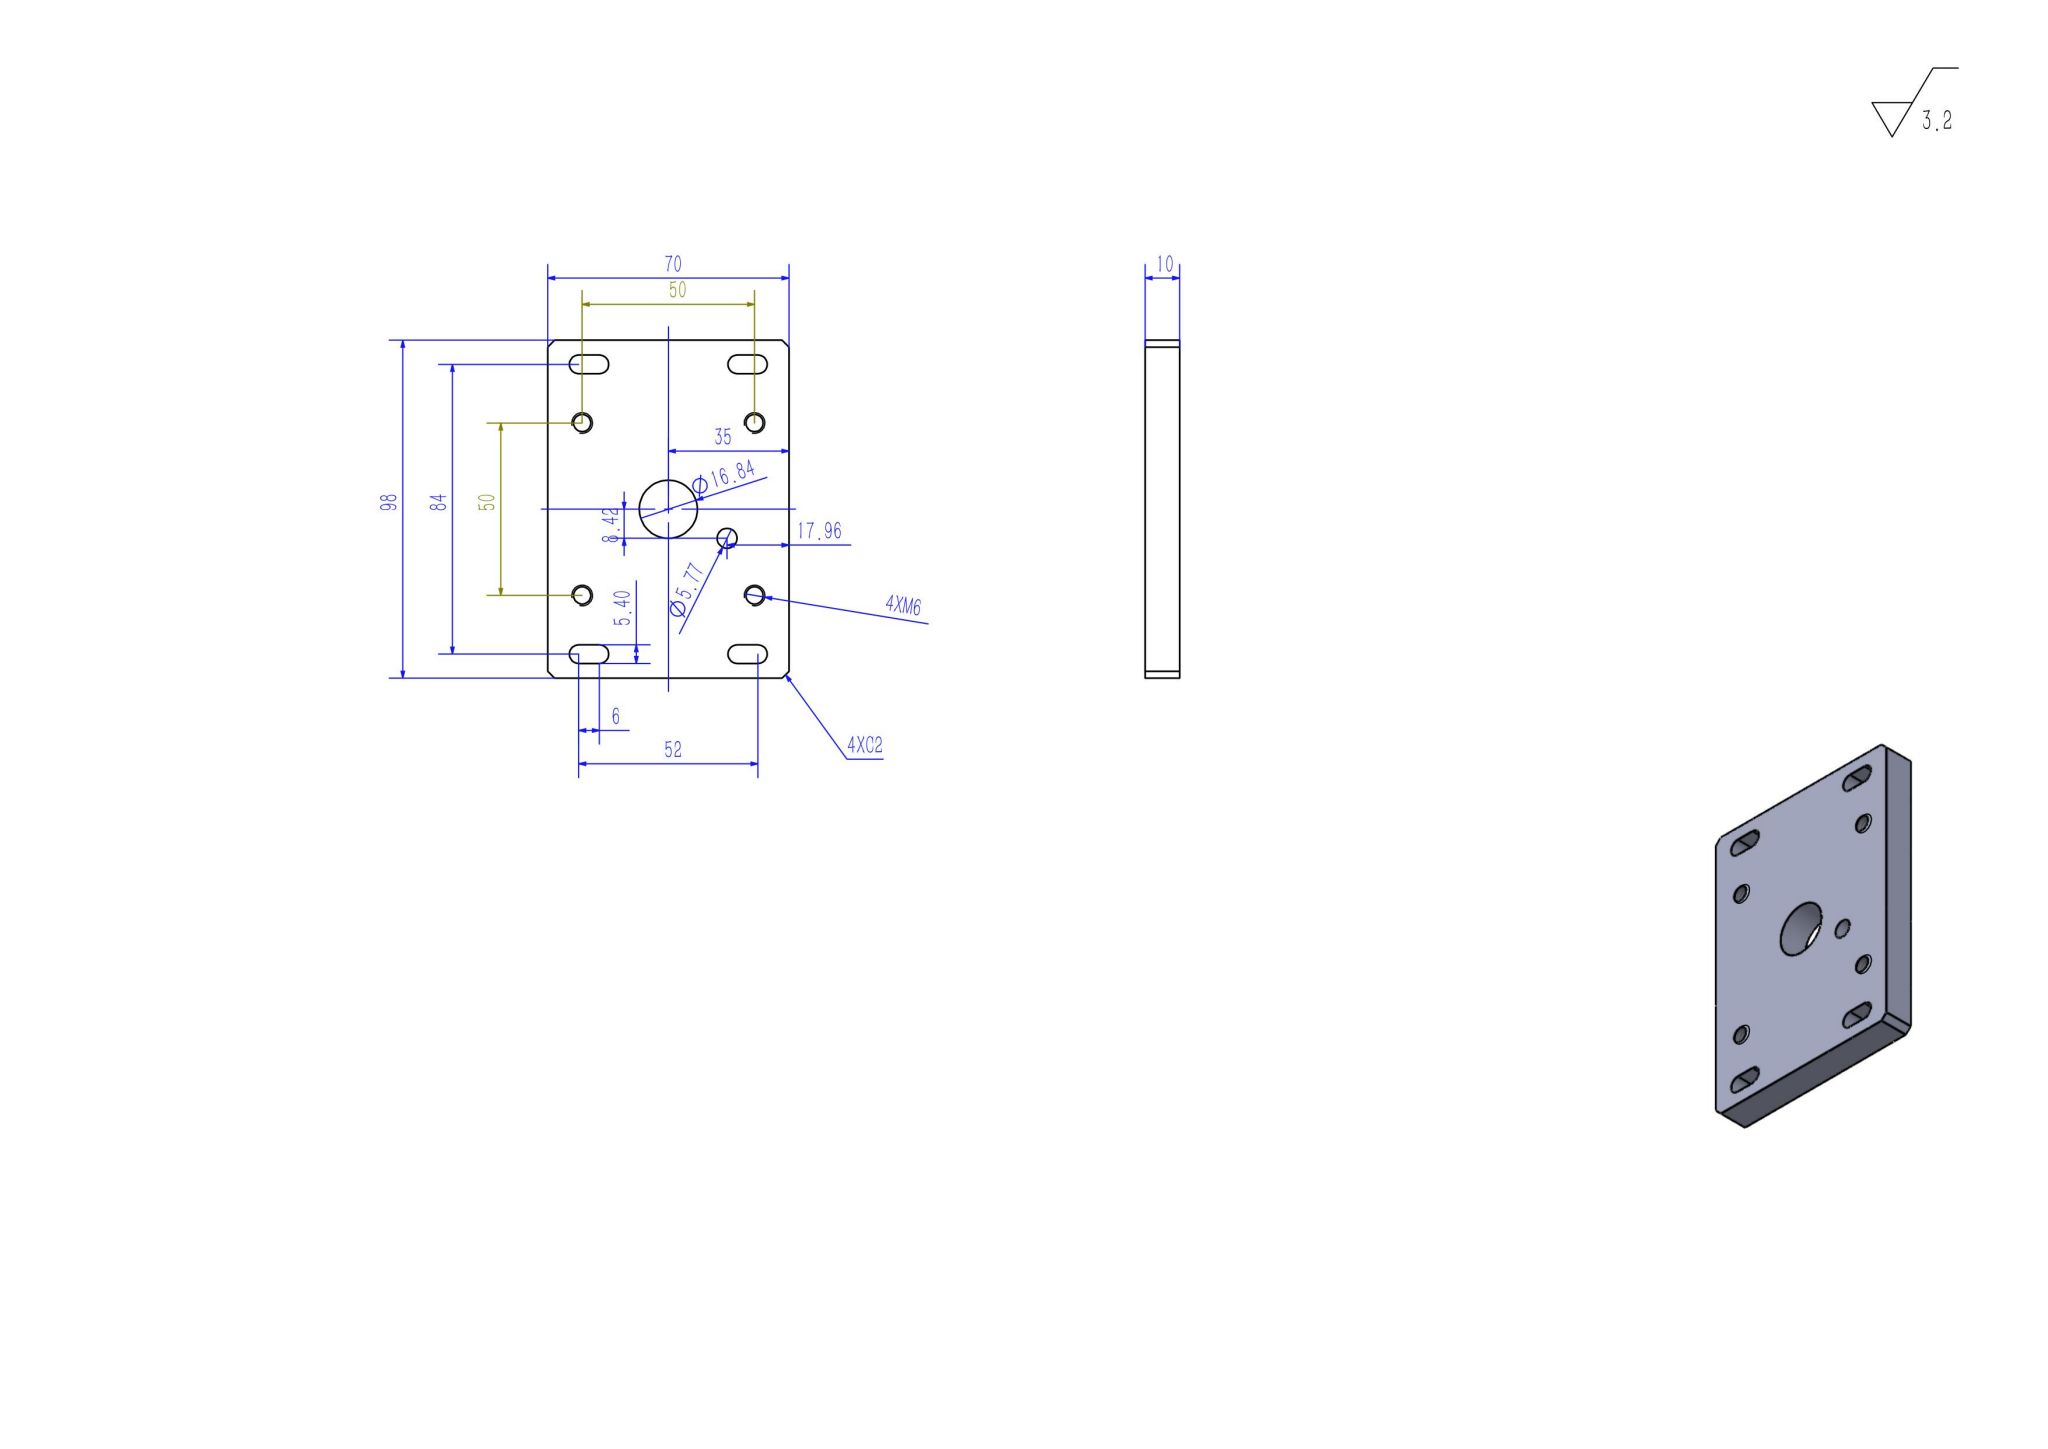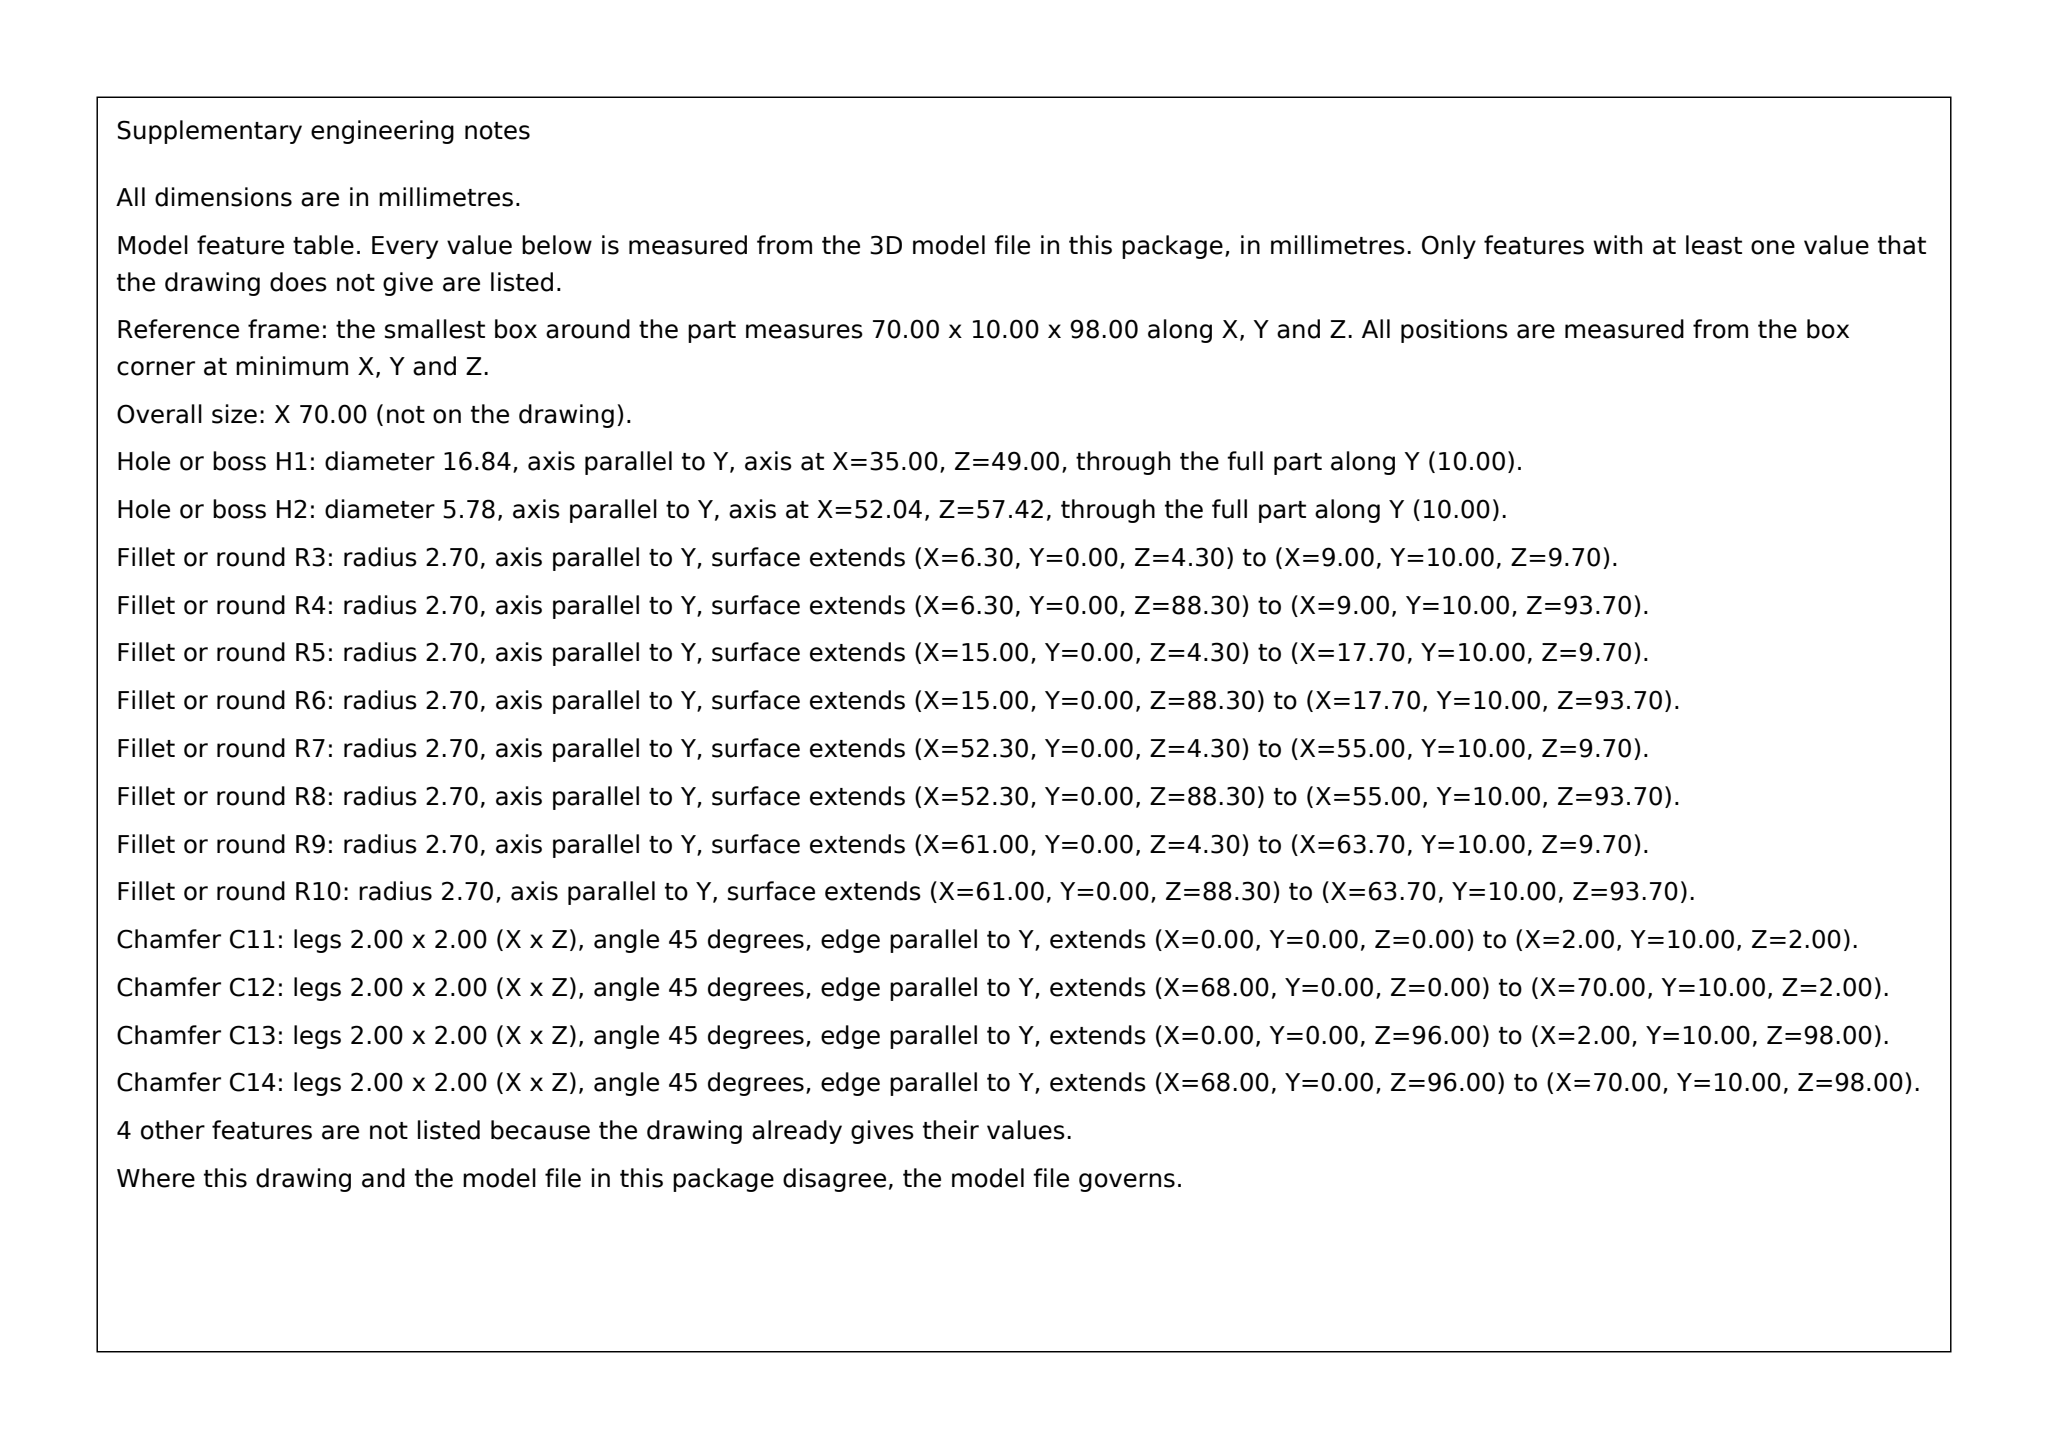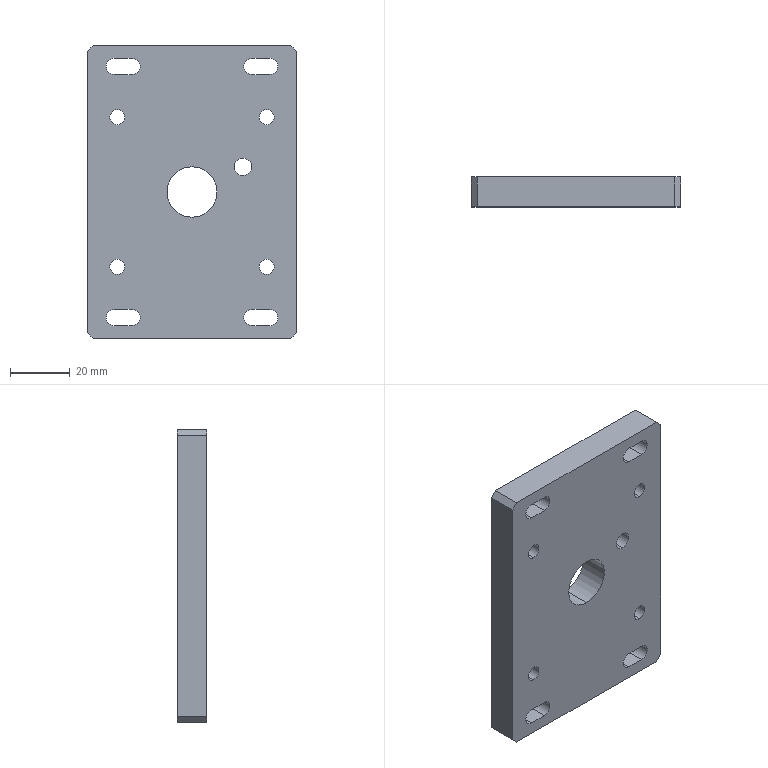Part | SolidWorks | mm | 1 solid | 38 faces | box 70 x 10 x 98 mm | volume 63034 mm3 | cylinder 20 | plane 18 | commonest cylinder face diameters 5 x8 5.4 x8 16.839 x2 5.77 x2
build123d program:
from build123d import *

# Parameters (mm, degrees)
SKETCH1_W             = 70
SKETCH1_H             = 98
BOSS_EXTRUDE1_DEPTH   = 10
M6_TAPPED_HOLE1_D     = 5
M6_TAPPED_HOLE1_DEPTH = 15
M6_TAPPED_HOLE1_TIP   = 1.502
CUT_EXTRUDE1_DEPTH    = 16
CHAMFER1_SIZE         = 2
SKETCH5_R             = 8.42
SKETCH5_R_2           = 2.885
CUT_EXTRUDE2_DEPTH    = 80


with BuildPart() as part:
    # Sketch1 → Boss-Extrude1 (new body)
    with BuildSketch(Plane(origin=(0, 0, 0), x_dir=(1, 0, 0), z_dir=(0, 1, 0))):
        Rectangle(SKETCH1_W, SKETCH1_H)
    extrude(amount=BOSS_EXTRUDE1_DEPTH)

    # M6 Tapped Hole1
    with Locations(Plane(origin=(0, 10, 0), x_dir=(1, 0, 0), z_dir=(0, 1, 0))):
        with Locations((25, 25), (-25, 25), (-25, -25), (25, -25)):
            Hole(M6_TAPPED_HOLE1_D / 2, depth=M6_TAPPED_HOLE1_DEPTH)
            with Locations((0, 0, -(M6_TAPPED_HOLE1_DEPTH + M6_TAPPED_HOLE1_TIP / 2))):  # 118° drill point
                Cone(0, M6_TAPPED_HOLE1_D / 2, M6_TAPPED_HOLE1_TIP, mode=Mode.SUBTRACT)

    # Sketch4 → Cut-Extrude1 (cut)
    with BuildSketch(Plane(origin=(0, 10, 0), x_dir=(1, 0, 0), z_dir=(0, 1, 0))):
        with BuildLine():
            Line((26, 39.3), (20, 39.3))
            ThreePointArc((20, 39.3), (17.3, 42), (20, 44.7))
            Line((20, 44.7), (26, 44.7))
            ThreePointArc((26, 44.7), (28.7, 42), (26, 39.3))
        make_face()
        with BuildLine():
            Line((-26, 39.3), (-20, 39.3))
            ThreePointArc((-20, 39.3), (-17.3, 42), (-20, 44.7))
            Line((-20, 44.7), (-26, 44.7))
            ThreePointArc((-26, 44.7), (-28.7, 42), (-26, 39.3))
        make_face()
        with BuildLine():
            Line((26, -39.3), (20, -39.3))
            ThreePointArc((20, -39.3), (17.3, -42), (20, -44.7))
            Line((20, -44.7), (26, -44.7))
            ThreePointArc((26, -44.7), (28.7, -42), (26, -39.3))
        make_face()
        with BuildLine():
            Line((-26, -39.3), (-20, -39.3))
            ThreePointArc((-20, -39.3), (-17.3, -42), (-20, -44.7))
            Line((-20, -44.7), (-26, -44.7))
            ThreePointArc((-26, -44.7), (-28.7, -42), (-26, -39.3))
        make_face()
    extrude(amount=-CUT_EXTRUDE1_DEPTH, mode=Mode.SUBTRACT)

    # Chamfer1
    chamfer1_edges = [part.edges().sort_by_distance(p)[0] for p in [
        (35, 5, 49),
        (-35, 5, 49),
        (-35, 5, -49),
        (35, 5, -49),
    ]]
    chamfer(chamfer1_edges, length=CHAMFER1_SIZE)

    # Sketch5 → Cut-Extrude2 (cut)
    with BuildSketch(Plane(origin=(0, 10, 0), x_dir=(1, 0, 0), z_dir=(0, 1, 0))):
        with Locations(Location((0, 0, 0), (0, 0, 270))):
            Circle(SKETCH5_R)
        with Locations(Location((17.039, -8.42, 0), (0, 0, 270))):
            Circle(SKETCH5_R_2)
    extrude(amount=-CUT_EXTRUDE2_DEPTH, mode=Mode.SUBTRACT)


solid = part.part